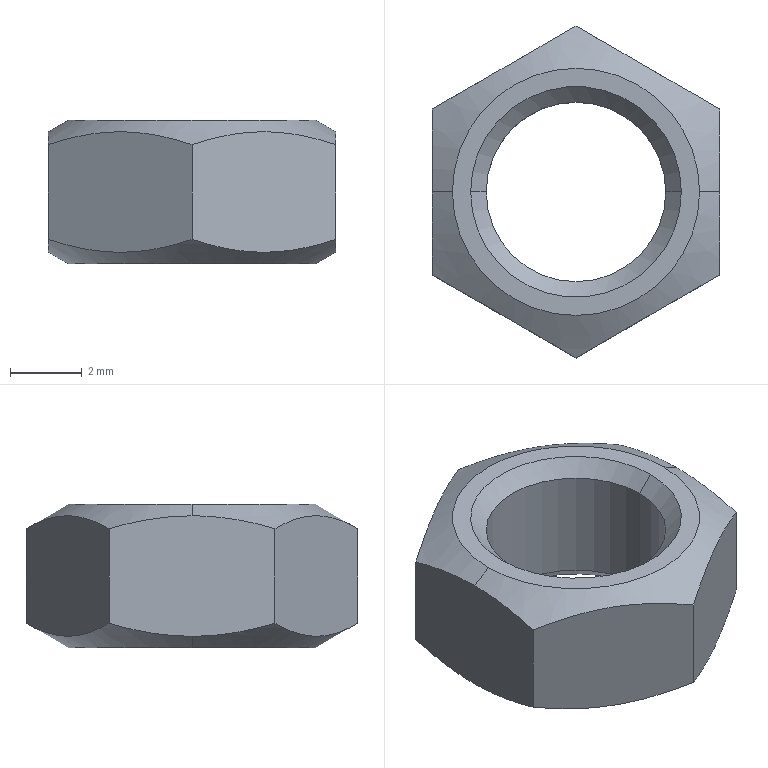Component | SolidWorks | F-YBCJ2_NTJ-015A-1 | 1 solid | 18 faces | box 8 x 9.24 x 4 mm | volume 131 mm3 | cone 8 | plane 8 | cylinder 2 | commonest cylinder face diameters 5 x2
build123d program:
from build123d import *

# Parameters (mm, degrees)
BOSS_EXTRUDE1_DEPTH      = 2
BOSS_EXTRUDE1_DEPTH_BACK = 2


with BuildPart() as part:
    # Sketch1 → Boss-Extrude1 (new, two sides: drawn at the far end of the back side and taken through both)
    with BuildSketch(Plane(origin=(0, 0, 0), x_dir=(0, 0, -1), z_dir=(1, 0, 0)).offset(-BOSS_EXTRUDE1_DEPTH_BACK)):
        Polygon((-4, 2.309), (-4, -2.309), (0, -4.619), (4, -2.309), (4, 2.309), (0, 4.619), align=None)
    extrude(amount=BOSS_EXTRUDE1_DEPTH + BOSS_EXTRUDE1_DEPTH_BACK)

    # Sketch2 → Cut-Revolve1 (revolve, cut)
    with BuildSketch(Plane.XY, mode=Mode.PRIVATE) as cut_revolve1_sk:
        Polygon((-2, 0), (-2, 2.933), (-1.567, 2.5), (1.567, 2.5), (2, 2.933), (2, 0), align=None)
    revolve(cut_revolve1_sk.sketch.rotate(Axis((2, 0, 0), (-1, 0, 0)), 270), axis=Axis((2, 0, 0), (-1, 0, 0)), mode=Mode.SUBTRACT)

    # Sketch3 → Cut-Revolve2 (revolve, cut)
    with BuildSketch(Plane.XY, mode=Mode.PRIVATE) as cut_revolve2_sk:
        Polygon((-7, 8.44), (-7, 1), (-2, 1), (-2, 3.44), (0, 6.904), (2, 3.44), (2, 1), (7, 1), (7, 8.44), align=None)
    revolve(cut_revolve2_sk.sketch.rotate(Axis((50, 0, 0), (-1, 0, 0)), 270), axis=Axis((50, 0, 0), (-1, 0, 0)), mode=Mode.SUBTRACT)


solid = part.part

# Placed as in the assembly
solid = solid.moved(Location((272.305, 302.175, 114.479), (0, 90, 0)))
STEP:
#1=COLOUR_RGB('',0.7922,0.8196,0.9333);
#2=FILL_AREA_STYLE_COLOUR('',#1);
#3=FILL_AREA_STYLE('',(#2));
#4=SURFACE_STYLE_FILL_AREA(#3);
#5=SURFACE_SIDE_STYLE('',(#4));
#6=SURFACE_STYLE_USAGE(.BOTH.,#5);
#7=PRESENTATION_STYLE_ASSIGNMENT((#6));
#8=CARTESIAN_POINT('',(10.856,11.897,4.586));
#9=VERTEX_POINT('',#8);
#10=CARTESIAN_POINT('',(10.585,11.897,4.586));
#11=VERTEX_POINT('',#10);
#12=CARTESIAN_POINT('',(10.721,11.897,4.586));
#13=DIRECTION('',(-0.,0.,1.));
#14=DIRECTION('',(1.,0.,0.));
#15=AXIS2_PLACEMENT_3D('',#12,#13,#14);
#16=CIRCLE('',#15,0.1354);
#17=EDGE_CURVE('',#9,#11,#16,.T.);
#18=ORIENTED_EDGE('',*,*,#17,.F.);
#19=CARTESIAN_POINT('',(10.878,11.897,4.573));
#20=VERTEX_POINT('',#19);
#21=CARTESIAN_POINT('',(10.856,11.897,4.586));
#22=DIRECTION('',(0.866,0.,-0.5));
#23=VECTOR('',#22,39.37);
#24=LINE('',#21,#23);
#25=EDGE_CURVE('',#9,#20,#24,.T.);
#26=ORIENTED_EDGE('',*,*,#25,.T.);
#27=CARTESIAN_POINT('',(10.878,11.988,4.559));
#28=VERTEX_POINT('',#27);
#29=CARTESIAN_POINT('',(10.878,11.897,4.573));
#30=CARTESIAN_POINT('',(10.878,11.912,4.573));
#31=CARTESIAN_POINT('',(10.878,11.928,4.572));
#32=CARTESIAN_POINT('',(10.878,11.958,4.567));
#33=CARTESIAN_POINT('',(10.878,11.973,4.563));
#34=CARTESIAN_POINT('',(10.878,11.988,4.559));
#35=B_SPLINE_CURVE_WITH_KNOTS('',3,(#29,#30,#31,#32,#33,#34),.UNSPECIFIED.,.F.,.F.,(4,2,4),(0.006456,0.007625,0.008794),.UNSPECIFIED.);
#36=EDGE_CURVE('',#20,#28,#35,.T.);
#37=ORIENTED_EDGE('',*,*,#36,.T.);
#38=CARTESIAN_POINT('',(10.721,12.079,4.559));
#39=VERTEX_POINT('',#38);
#40=CARTESIAN_POINT('',(10.878,11.988,4.559));
#41=CARTESIAN_POINT('',(10.852,12.002,4.568));
#42=CARTESIAN_POINT('',(10.826,12.018,4.573));
#43=CARTESIAN_POINT('',(10.786,12.041,4.573));
#44=CARTESIAN_POINT('',(10.773,12.048,4.572));
#45=CARTESIAN_POINT('',(10.747,12.064,4.567));
#46=CARTESIAN_POINT('',(10.734,12.071,4.563));
#47=CARTESIAN_POINT('',(10.721,12.079,4.559));
#48=B_SPLINE_CURVE_WITH_KNOTS('',3,(#40,#41,#42,#43,#44,#45,#46,#47),.UNSPECIFIED.,.F.,.F.,(4,2,2,4),(0.00000024,0.002333,0.003499,0.004665),.UNSPECIFIED.);
#49=EDGE_CURVE('',#28,#39,#48,.T.);
#50=ORIENTED_EDGE('',*,*,#49,.T.);
#51=CARTESIAN_POINT('',(10.563,11.988,4.559));
#52=VERTEX_POINT('',#51);
#53=CARTESIAN_POINT('',(10.721,12.079,4.559));
#54=CARTESIAN_POINT('',(10.695,12.064,4.568));
#55=CARTESIAN_POINT('',(10.669,12.049,4.573));
#56=CARTESIAN_POINT('',(10.629,12.025,4.573));
#57=CARTESIAN_POINT('',(10.615,12.018,4.572));
#58=CARTESIAN_POINT('',(10.589,12.003,4.567));
#59=CARTESIAN_POINT('',(10.576,11.995,4.563));
#60=CARTESIAN_POINT('',(10.563,11.988,4.559));
#61=B_SPLINE_CURVE_WITH_KNOTS('',3,(#53,#54,#55,#56,#57,#58,#59,#60),.UNSPECIFIED.,.F.,.F.,(4,2,2,4),(0.00000024,0.002333,0.003499,0.004665),.UNSPECIFIED.);
#62=EDGE_CURVE('',#39,#52,#61,.T.);
#63=ORIENTED_EDGE('',*,*,#62,.T.);
#64=CARTESIAN_POINT('',(10.563,11.897,4.573));
#65=VERTEX_POINT('',#64);
#66=CARTESIAN_POINT('',(10.563,11.988,4.559));
#67=CARTESIAN_POINT('',(10.563,11.973,4.563));
#68=CARTESIAN_POINT('',(10.563,11.958,4.567));
#69=CARTESIAN_POINT('',(10.563,11.928,4.572));
#70=CARTESIAN_POINT('',(10.563,11.912,4.573));
#71=CARTESIAN_POINT('',(10.563,11.897,4.573));
#72=B_SPLINE_CURVE_WITH_KNOTS('',3,(#66,#67,#68,#69,#70,#71),.UNSPECIFIED.,.F.,.F.,(4,2,4),(0.01181,0.01298,0.01415),.UNSPECIFIED.);
#73=EDGE_CURVE('',#52,#65,#72,.T.);
#74=ORIENTED_EDGE('',*,*,#73,.T.);
#75=CARTESIAN_POINT('',(10.585,11.897,4.586));
#76=DIRECTION('',(-0.866,0.,-0.5));
#77=VECTOR('',#76,39.37);
#78=LINE('',#75,#77);
#79=EDGE_CURVE('',#11,#65,#78,.T.);
#80=ORIENTED_EDGE('',*,*,#79,.F.);
#81=EDGE_LOOP('',(#18,#26,#37,#50,#63,#74,#80));
#82=FACE_OUTER_BOUND('',#81,.T.);
#83=CARTESIAN_POINT('',(10.721,11.897,4.586));
#84=DIRECTION('',(0.,-0.,-1.));
#85=DIRECTION('',(-1.,0.,0.));
#86=AXIS2_PLACEMENT_3D('',#83,#84,#85);
#87=CONICAL_SURFACE('',#86,0.1354,1.047);
#88=ADVANCED_FACE('',(#82),#87,.T.);
#89=CARTESIAN_POINT('',(10.856,11.897,4.428));
#90=VERTEX_POINT('',#89);
#91=CARTESIAN_POINT('',(10.585,11.897,4.428));
#92=VERTEX_POINT('',#91);
#93=CARTESIAN_POINT('',(10.721,11.897,4.428));
#94=DIRECTION('',(-0.,0.,1.));
#95=DIRECTION('',(1.,0.,0.));
#96=AXIS2_PLACEMENT_3D('',#93,#94,#95);
#97=CIRCLE('',#96,0.1354);
#98=EDGE_CURVE('',#90,#92,#97,.T.);
#99=ORIENTED_EDGE('',*,*,#98,.T.);
#100=CARTESIAN_POINT('',(10.563,11.897,4.441));
#101=VERTEX_POINT('',#100);
#102=CARTESIAN_POINT('',(10.449,11.897,4.507));
#103=DIRECTION('',(-0.866,0.,0.5));
#104=VECTOR('',#103,39.37);
#105=LINE('',#102,#104);
#106=EDGE_CURVE('',#92,#101,#105,.T.);
#107=ORIENTED_EDGE('',*,*,#106,.T.);
#108=CARTESIAN_POINT('',(10.563,11.988,4.455));
#109=VERTEX_POINT('',#108);
#110=CARTESIAN_POINT('',(10.563,11.897,4.441));
#111=CARTESIAN_POINT('',(10.563,11.912,4.441));
#112=CARTESIAN_POINT('',(10.563,11.928,4.442));
#113=CARTESIAN_POINT('',(10.563,11.958,4.447));
#114=CARTESIAN_POINT('',(10.563,11.973,4.451));
#115=CARTESIAN_POINT('',(10.563,11.988,4.455));
#116=B_SPLINE_CURVE_WITH_KNOTS('',3,(#110,#111,#112,#113,#114,#115),.UNSPECIFIED.,.F.,.F.,(4,2,4),(0.006456,0.007625,0.008794),.UNSPECIFIED.);
#117=EDGE_CURVE('',#101,#109,#116,.T.);
#118=ORIENTED_EDGE('',*,*,#117,.T.);
#119=CARTESIAN_POINT('',(10.721,12.079,4.455));
#120=VERTEX_POINT('',#119);
#121=CARTESIAN_POINT('',(10.563,11.988,4.455));
#122=CARTESIAN_POINT('',(10.589,12.002,4.447));
#123=CARTESIAN_POINT('',(10.615,12.018,4.441));
#124=CARTESIAN_POINT('',(10.655,12.041,4.441));
#125=CARTESIAN_POINT('',(10.669,12.048,4.442));
#126=CARTESIAN_POINT('',(10.695,12.064,4.447));
#127=CARTESIAN_POINT('',(10.708,12.071,4.451));
#128=CARTESIAN_POINT('',(10.721,12.079,4.455));
#129=B_SPLINE_CURVE_WITH_KNOTS('',3,(#121,#122,#123,#124,#125,#126,#127,#128),.UNSPECIFIED.,.F.,.F.,(4,2,2,4),(0.00000024,0.002333,0.003499,0.004665),.UNSPECIFIED.);
#130=EDGE_CURVE('',#109,#120,#129,.T.);
#131=ORIENTED_EDGE('',*,*,#130,.T.);
#132=CARTESIAN_POINT('',(10.878,11.988,4.455));
#133=VERTEX_POINT('',#132);
#134=CARTESIAN_POINT('',(10.721,12.079,4.455));
#135=CARTESIAN_POINT('',(10.746,12.064,4.447));
#136=CARTESIAN_POINT('',(10.772,12.049,4.441));
#137=CARTESIAN_POINT('',(10.813,12.025,4.441));
#138=CARTESIAN_POINT('',(10.826,12.018,4.442));
#139=CARTESIAN_POINT('',(10.852,12.003,4.447));
#140=CARTESIAN_POINT('',(10.865,11.995,4.451));
#141=CARTESIAN_POINT('',(10.878,11.988,4.455));
#142=B_SPLINE_CURVE_WITH_KNOTS('',3,(#134,#135,#136,#137,#138,#139,#140,#141),.UNSPECIFIED.,.F.,.F.,(4,2,2,4),(0.00000024,0.002333,0.003499,0.004665),.UNSPECIFIED.);
#143=EDGE_CURVE('',#120,#133,#142,.T.);
#144=ORIENTED_EDGE('',*,*,#143,.T.);
#145=CARTESIAN_POINT('',(10.878,11.897,4.441));
#146=VERTEX_POINT('',#145);
#147=CARTESIAN_POINT('',(10.878,11.988,4.455));
#148=CARTESIAN_POINT('',(10.878,11.973,4.451));
#149=CARTESIAN_POINT('',(10.878,11.958,4.447));
#150=CARTESIAN_POINT('',(10.878,11.928,4.442));
#151=CARTESIAN_POINT('',(10.878,11.912,4.441));
#152=CARTESIAN_POINT('',(10.878,11.897,4.441));
#153=B_SPLINE_CURVE_WITH_KNOTS('',3,(#147,#148,#149,#150,#151,#152),.UNSPECIFIED.,.F.,.F.,(4,2,4),(0.01181,0.01298,0.01415),.UNSPECIFIED.);
#154=EDGE_CURVE('',#133,#146,#153,.T.);
#155=ORIENTED_EDGE('',*,*,#154,.T.);
#156=CARTESIAN_POINT('',(10.992,11.897,4.507));
#157=DIRECTION('',(0.866,-0.,0.5));
#158=VECTOR('',#157,39.37);
#159=LINE('',#156,#158);
#160=EDGE_CURVE('',#90,#146,#159,.T.);
#161=ORIENTED_EDGE('',*,*,#160,.F.);
#162=EDGE_LOOP('',(#99,#107,#118,#131,#144,#155,#161));
#163=FACE_OUTER_BOUND('',#162,.T.);
#164=CARTESIAN_POINT('',(10.721,11.897,4.507));
#165=DIRECTION('',(-0.,0.,1.));
#166=DIRECTION('',(1.,0.,0.));
#167=AXIS2_PLACEMENT_3D('',#164,#165,#166);
#168=CONICAL_SURFACE('',#167,0.2718,1.047);
#169=ADVANCED_FACE('',(#163),#168,.T.);
#170=CARTESIAN_POINT('',(10.622,11.897,4.445));
#171=VERTEX_POINT('',#170);
#172=CARTESIAN_POINT('',(10.819,11.897,4.445));
#173=VERTEX_POINT('',#172);
#174=CARTESIAN_POINT('',(10.721,11.897,4.445));
#175=DIRECTION('',(-0.,0.,1.));
#176=DIRECTION('',(1.,0.,0.));
#177=AXIS2_PLACEMENT_3D('',#174,#175,#176);
#178=CIRCLE('',#177,0.09843);
#179=EDGE_CURVE('',#171,#173,#178,.T.);
#180=ORIENTED_EDGE('',*,*,#179,.T.);
#181=CARTESIAN_POINT('',(10.836,11.897,4.428));
#182=VERTEX_POINT('',#181);
#183=CARTESIAN_POINT('',(10.836,11.897,4.428));
#184=DIRECTION('',(0.7071,0.,-0.7071));
#185=VECTOR('',#184,39.37);
#186=LINE('',#183,#185);
#187=EDGE_CURVE('',#173,#182,#186,.T.);
#188=ORIENTED_EDGE('',*,*,#187,.T.);
#189=CARTESIAN_POINT('',(10.605,11.897,4.428));
#190=VERTEX_POINT('',#189);
#191=CARTESIAN_POINT('',(10.721,11.897,4.428));
#192=DIRECTION('',(-0.,0.,1.));
#193=DIRECTION('',(1.,0.,0.));
#194=AXIS2_PLACEMENT_3D('',#191,#192,#193);
#195=CIRCLE('',#194,0.1155);
#196=EDGE_CURVE('',#190,#182,#195,.T.);
#197=ORIENTED_EDGE('',*,*,#196,.F.);
#198=CARTESIAN_POINT('',(10.605,11.897,4.428));
#199=DIRECTION('',(-0.7071,-0.,-0.7071));
#200=VECTOR('',#199,39.37);
#201=LINE('',#198,#200);
#202=EDGE_CURVE('',#171,#190,#201,.T.);
#203=ORIENTED_EDGE('',*,*,#202,.F.);
#204=EDGE_LOOP('',(#180,#188,#197,#203));
#205=FACE_OUTER_BOUND('',#204,.T.);
#206=CARTESIAN_POINT('',(10.721,11.897,4.428));
#207=DIRECTION('',(0.,-0.,-1.));
#208=DIRECTION('',(-1.,0.,0.));
#209=AXIS2_PLACEMENT_3D('',#206,#207,#208);
#210=CONICAL_SURFACE('',#209,0.1155,0.7854);
#211=ADVANCED_FACE('',(#205),#210,.F.);
#212=ORIENTED_EDGE('',*,*,#179,.F.);
#213=CARTESIAN_POINT('',(10.622,11.897,4.569));
#214=VERTEX_POINT('',#213);
#215=CARTESIAN_POINT('',(10.622,11.897,4.428));
#216=DIRECTION('',(-0.,0.,1.));
#217=VECTOR('',#216,39.37);
#218=LINE('',#215,#217);
#219=EDGE_CURVE('',#171,#214,#218,.T.);
#220=ORIENTED_EDGE('',*,*,#219,.T.);
#221=CARTESIAN_POINT('',(10.819,11.897,4.569));
#222=VERTEX_POINT('',#221);
#223=CARTESIAN_POINT('',(10.721,11.897,4.569));
#224=DIRECTION('',(-0.,0.,1.));
#225=DIRECTION('',(1.,0.,0.));
#226=AXIS2_PLACEMENT_3D('',#223,#224,#225);
#227=CIRCLE('',#226,0.09843);
#228=EDGE_CURVE('',#214,#222,#227,.T.);
#229=ORIENTED_EDGE('',*,*,#228,.T.);
#230=CARTESIAN_POINT('',(10.819,11.897,4.428));
#231=DIRECTION('',(-0.,0.,1.));
#232=VECTOR('',#231,39.37);
#233=LINE('',#230,#232);
#234=EDGE_CURVE('',#173,#222,#233,.T.);
#235=ORIENTED_EDGE('',*,*,#234,.F.);
#236=EDGE_LOOP('',(#212,#220,#229,#235));
#237=FACE_OUTER_BOUND('',#236,.T.);
#238=CARTESIAN_POINT('',(10.721,11.897,4.428));
#239=DIRECTION('',(-0.,0.,1.));
#240=DIRECTION('',(1.,0.,0.));
#241=AXIS2_PLACEMENT_3D('',#238,#239,#240);
#242=CYLINDRICAL_SURFACE('',#241,0.09843);
#243=ADVANCED_FACE('',(#237),#242,.F.);
#244=ORIENTED_EDGE('',*,*,#228,.F.);
#245=CARTESIAN_POINT('',(10.605,11.897,4.586));
#246=VERTEX_POINT('',#245);
#247=CARTESIAN_POINT('',(10.622,11.897,4.569));
#248=DIRECTION('',(-0.7071,0.,0.7071));
#249=VECTOR('',#248,39.37);
#250=LINE('',#247,#249);
#251=EDGE_CURVE('',#214,#246,#250,.T.);
#252=ORIENTED_EDGE('',*,*,#251,.T.);
#253=CARTESIAN_POINT('',(10.836,11.897,4.586));
#254=VERTEX_POINT('',#253);
#255=CARTESIAN_POINT('',(10.721,11.897,4.586));
#256=DIRECTION('',(-0.,0.,1.));
#257=DIRECTION('',(1.,0.,0.));
#258=AXIS2_PLACEMENT_3D('',#255,#256,#257);
#259=CIRCLE('',#258,0.1155);
#260=EDGE_CURVE('',#246,#254,#259,.T.);
#261=ORIENTED_EDGE('',*,*,#260,.T.);
#262=CARTESIAN_POINT('',(10.819,11.897,4.569));
#263=DIRECTION('',(0.7071,0.,0.7071));
#264=VECTOR('',#263,39.37);
#265=LINE('',#262,#264);
#266=EDGE_CURVE('',#222,#254,#265,.T.);
#267=ORIENTED_EDGE('',*,*,#266,.F.);
#268=EDGE_LOOP('',(#244,#252,#261,#267));
#269=FACE_OUTER_BOUND('',#268,.T.);
#270=CARTESIAN_POINT('',(10.721,11.897,4.569));
#271=DIRECTION('',(-0.,0.,1.));
#272=DIRECTION('',(1.,0.,0.));
#273=AXIS2_PLACEMENT_3D('',#270,#271,#272);
#274=CONICAL_SURFACE('',#273,0.09843,0.7854);
#275=ADVANCED_FACE('',(#269),#274,.F.);
#276=ORIENTED_EDGE('',*,*,#196,.T.);
#277=CARTESIAN_POINT('',(10.721,11.897,4.428));
#278=DIRECTION('',(-0.,0.,1.));
#279=DIRECTION('',(1.,0.,0.));
#280=AXIS2_PLACEMENT_3D('',#277,#278,#279);
#281=CIRCLE('',#280,0.1155);
#282=EDGE_CURVE('',#182,#190,#281,.T.);
#283=ORIENTED_EDGE('',*,*,#282,.T.);
#284=EDGE_LOOP('',(#276,#283));
#285=FACE_BOUND('',#284,.T.);
#286=ORIENTED_EDGE('',*,*,#98,.F.);
#287=CARTESIAN_POINT('',(10.721,11.897,4.428));
#288=DIRECTION('',(-0.,0.,1.));
#289=DIRECTION('',(1.,0.,0.));
#290=AXIS2_PLACEMENT_3D('',#287,#288,#289);
#291=CIRCLE('',#290,0.1354);
#292=EDGE_CURVE('',#92,#90,#291,.T.);
#293=ORIENTED_EDGE('',*,*,#292,.F.);
#294=EDGE_LOOP('',(#286,#293));
#295=FACE_OUTER_BOUND('',#294,.T.);
#296=CARTESIAN_POINT('',(10.721,11.897,4.428));
#297=DIRECTION('',(0.,-0.,-1.));
#298=DIRECTION('',(-1.,0.,-0.));
#299=AXIS2_PLACEMENT_3D('',#296,#297,#298);
#300=PLANE('',#299);
#301=ADVANCED_FACE('',(#285,#295),#300,.T.);
#302=CARTESIAN_POINT('',(10.721,11.897,4.586));
#303=DIRECTION('',(-0.,0.,1.));
#304=DIRECTION('',(1.,0.,0.));
#305=AXIS2_PLACEMENT_3D('',#302,#303,#304);
#306=CIRCLE('',#305,0.1155);
#307=EDGE_CURVE('',#254,#246,#306,.T.);
#308=ORIENTED_EDGE('',*,*,#307,.F.);
#309=ORIENTED_EDGE('',*,*,#260,.F.);
#310=EDGE_LOOP('',(#308,#309));
#311=FACE_BOUND('',#310,.T.);
#312=CARTESIAN_POINT('',(10.721,11.897,4.586));
#313=DIRECTION('',(-0.,0.,1.));
#314=DIRECTION('',(1.,0.,0.));
#315=AXIS2_PLACEMENT_3D('',#312,#313,#314);
#316=CIRCLE('',#315,0.1354);
#317=EDGE_CURVE('',#11,#9,#316,.T.);
#318=ORIENTED_EDGE('',*,*,#317,.T.);
#319=ORIENTED_EDGE('',*,*,#17,.T.);
#320=EDGE_LOOP('',(#318,#319));
#321=FACE_OUTER_BOUND('',#320,.T.);
#322=CARTESIAN_POINT('',(10.721,11.897,4.586));
#323=DIRECTION('',(0.,-0.,-1.));
#324=DIRECTION('',(-1.,0.,-0.));
#325=AXIS2_PLACEMENT_3D('',#322,#323,#324);
#326=PLANE('',#325);
#327=ADVANCED_FACE('',(#311,#321),#326,.F.);
#328=ORIENTED_EDGE('',*,*,#251,.F.);
#329=CARTESIAN_POINT('',(10.721,11.897,4.569));
#330=DIRECTION('',(-0.,0.,1.));
#331=DIRECTION('',(1.,0.,0.));
#332=AXIS2_PLACEMENT_3D('',#329,#330,#331);
#333=CIRCLE('',#332,0.09843);
#334=EDGE_CURVE('',#222,#214,#333,.T.);
#335=ORIENTED_EDGE('',*,*,#334,.F.);
#336=ORIENTED_EDGE('',*,*,#266,.T.);
#337=ORIENTED_EDGE('',*,*,#307,.T.);
#338=EDGE_LOOP('',(#328,#335,#336,#337));
#339=FACE_OUTER_BOUND('',#338,.T.);
#340=CARTESIAN_POINT('',(10.721,11.897,4.569));
#341=DIRECTION('',(-0.,0.,1.));
#342=DIRECTION('',(1.,0.,0.));
#343=AXIS2_PLACEMENT_3D('',#340,#341,#342);
#344=CONICAL_SURFACE('',#343,0.09843,0.7854);
#345=ADVANCED_FACE('',(#339),#344,.F.);
#346=ORIENTED_EDGE('',*,*,#219,.F.);
#347=CARTESIAN_POINT('',(10.721,11.897,4.445));
#348=DIRECTION('',(-0.,0.,1.));
#349=DIRECTION('',(1.,0.,0.));
#350=AXIS2_PLACEMENT_3D('',#347,#348,#349);
#351=CIRCLE('',#350,0.09843);
#352=EDGE_CURVE('',#173,#171,#351,.T.);
#353=ORIENTED_EDGE('',*,*,#352,.F.);
#354=ORIENTED_EDGE('',*,*,#234,.T.);
#355=ORIENTED_EDGE('',*,*,#334,.T.);
#356=EDGE_LOOP('',(#346,#353,#354,#355));
#357=FACE_OUTER_BOUND('',#356,.T.);
#358=CARTESIAN_POINT('',(10.721,11.897,4.428));
#359=DIRECTION('',(-0.,0.,1.));
#360=DIRECTION('',(1.,0.,0.));
#361=AXIS2_PLACEMENT_3D('',#358,#359,#360);
#362=CYLINDRICAL_SURFACE('',#361,0.09843);
#363=ADVANCED_FACE('',(#357),#362,.F.);
#364=ORIENTED_EDGE('',*,*,#187,.F.);
#365=ORIENTED_EDGE('',*,*,#352,.T.);
#366=ORIENTED_EDGE('',*,*,#202,.T.);
#367=ORIENTED_EDGE('',*,*,#282,.F.);
#368=EDGE_LOOP('',(#364,#365,#366,#367));
#369=FACE_OUTER_BOUND('',#368,.T.);
#370=CARTESIAN_POINT('',(10.721,11.897,4.428));
#371=DIRECTION('',(0.,-0.,-1.));
#372=DIRECTION('',(-1.,0.,0.));
#373=AXIS2_PLACEMENT_3D('',#370,#371,#372);
#374=CONICAL_SURFACE('',#373,0.1155,0.7854);
#375=ADVANCED_FACE('',(#369),#374,.F.);
#376=ORIENTED_EDGE('',*,*,#106,.F.);
#377=ORIENTED_EDGE('',*,*,#292,.T.);
#378=ORIENTED_EDGE('',*,*,#160,.T.);
#379=CARTESIAN_POINT('',(10.878,11.806,4.455));
#380=VERTEX_POINT('',#379);
#381=CARTESIAN_POINT('',(10.878,11.897,4.441));
#382=CARTESIAN_POINT('',(10.878,11.881,4.441));
#383=CARTESIAN_POINT('',(10.878,11.866,4.442));
#384=CARTESIAN_POINT('',(10.878,11.836,4.447));
#385=CARTESIAN_POINT('',(10.878,11.821,4.451));
#386=CARTESIAN_POINT('',(10.878,11.806,4.455));
#387=B_SPLINE_CURVE_WITH_KNOTS('',3,(#381,#382,#383,#384,#385,#386),.UNSPECIFIED.,.F.,.F.,(4,2,4),(0.01415,0.01532,0.01649),.UNSPECIFIED.);
#388=EDGE_CURVE('',#146,#380,#387,.T.);
#389=ORIENTED_EDGE('',*,*,#388,.T.);
#390=CARTESIAN_POINT('',(10.721,11.715,4.455));
#391=VERTEX_POINT('',#390);
#392=CARTESIAN_POINT('',(10.878,11.806,4.455));
#393=CARTESIAN_POINT('',(10.852,11.791,4.447));
#394=CARTESIAN_POINT('',(10.826,11.776,4.441));
#395=CARTESIAN_POINT('',(10.786,11.753,4.441));
#396=CARTESIAN_POINT('',(10.773,11.745,4.442));
#397=CARTESIAN_POINT('',(10.747,11.73,4.447));
#398=CARTESIAN_POINT('',(10.734,11.722,4.451));
#399=CARTESIAN_POINT('',(10.721,11.715,4.455));
#400=B_SPLINE_CURVE_WITH_KNOTS('',3,(#392,#393,#394,#395,#396,#397,#398,#399),.UNSPECIFIED.,.F.,.F.,(4,2,2,4),(0.00000024,0.002333,0.003499,0.004665),.UNSPECIFIED.);
#401=EDGE_CURVE('',#380,#391,#400,.T.);
#402=ORIENTED_EDGE('',*,*,#401,.T.);
#403=CARTESIAN_POINT('',(10.563,11.806,4.455));
#404=VERTEX_POINT('',#403);
#405=CARTESIAN_POINT('',(10.721,11.715,4.455));
#406=CARTESIAN_POINT('',(10.695,11.73,4.447));
#407=CARTESIAN_POINT('',(10.669,11.745,4.441));
#408=CARTESIAN_POINT('',(10.629,11.768,4.441));
#409=CARTESIAN_POINT('',(10.615,11.776,4.442));
#410=CARTESIAN_POINT('',(10.589,11.791,4.447));
#411=CARTESIAN_POINT('',(10.576,11.798,4.451));
#412=CARTESIAN_POINT('',(10.563,11.806,4.455));
#413=B_SPLINE_CURVE_WITH_KNOTS('',3,(#405,#406,#407,#408,#409,#410,#411,#412),.UNSPECIFIED.,.F.,.F.,(4,2,2,4),(0.00000024,0.002333,0.003499,0.004665),.UNSPECIFIED.);
#414=EDGE_CURVE('',#391,#404,#413,.T.);
#415=ORIENTED_EDGE('',*,*,#414,.T.);
#416=CARTESIAN_POINT('',(10.563,11.806,4.455));
#417=CARTESIAN_POINT('',(10.563,11.821,4.451));
#418=CARTESIAN_POINT('',(10.563,11.836,4.447));
#419=CARTESIAN_POINT('',(10.563,11.866,4.442));
#420=CARTESIAN_POINT('',(10.563,11.881,4.441));
#421=CARTESIAN_POINT('',(10.563,11.897,4.441));
#422=B_SPLINE_CURVE_WITH_KNOTS('',3,(#416,#417,#418,#419,#420,#421),.UNSPECIFIED.,.F.,.F.,(4,2,4),(0.00412,0.005288,0.006456),.UNSPECIFIED.);
#423=EDGE_CURVE('',#404,#101,#422,.T.);
#424=ORIENTED_EDGE('',*,*,#423,.T.);
#425=EDGE_LOOP('',(#376,#377,#378,#389,#402,#415,#424));
#426=FACE_OUTER_BOUND('',#425,.T.);
#427=CARTESIAN_POINT('',(10.721,11.897,4.507));
#428=DIRECTION('',(-0.,0.,1.));
#429=DIRECTION('',(1.,0.,0.));
#430=AXIS2_PLACEMENT_3D('',#427,#428,#429);
#431=CONICAL_SURFACE('',#430,0.2718,1.047);
#432=ADVANCED_FACE('',(#426),#431,.T.);
#433=ORIENTED_EDGE('',*,*,#25,.F.);
#434=ORIENTED_EDGE('',*,*,#317,.F.);
#435=ORIENTED_EDGE('',*,*,#79,.T.);
#436=CARTESIAN_POINT('',(10.563,11.806,4.559));
#437=VERTEX_POINT('',#436);
#438=CARTESIAN_POINT('',(10.563,11.897,4.573));
#439=CARTESIAN_POINT('',(10.563,11.881,4.573));
#440=CARTESIAN_POINT('',(10.563,11.866,4.572));
#441=CARTESIAN_POINT('',(10.563,11.836,4.567));
#442=CARTESIAN_POINT('',(10.563,11.821,4.563));
#443=CARTESIAN_POINT('',(10.563,11.806,4.559));
#444=B_SPLINE_CURVE_WITH_KNOTS('',3,(#438,#439,#440,#441,#442,#443),.UNSPECIFIED.,.F.,.F.,(4,2,4),(0.01415,0.01532,0.01649),.UNSPECIFIED.);
#445=EDGE_CURVE('',#65,#437,#444,.T.);
#446=ORIENTED_EDGE('',*,*,#445,.T.);
#447=CARTESIAN_POINT('',(10.721,11.715,4.559));
#448=VERTEX_POINT('',#447);
#449=CARTESIAN_POINT('',(10.563,11.806,4.559));
#450=CARTESIAN_POINT('',(10.589,11.791,4.568));
#451=CARTESIAN_POINT('',(10.615,11.776,4.573));
#452=CARTESIAN_POINT('',(10.655,11.753,4.573));
#453=CARTESIAN_POINT('',(10.669,11.745,4.572));
#454=CARTESIAN_POINT('',(10.695,11.73,4.567));
#455=CARTESIAN_POINT('',(10.708,11.722,4.563));
#456=CARTESIAN_POINT('',(10.721,11.715,4.559));
#457=B_SPLINE_CURVE_WITH_KNOTS('',3,(#449,#450,#451,#452,#453,#454,#455,#456),.UNSPECIFIED.,.F.,.F.,(4,2,2,4),(0.00000024,0.002333,0.003499,0.004665),.UNSPECIFIED.);
#458=EDGE_CURVE('',#437,#448,#457,.T.);
#459=ORIENTED_EDGE('',*,*,#458,.T.);
#460=CARTESIAN_POINT('',(10.878,11.806,4.559));
#461=VERTEX_POINT('',#460);
#462=CARTESIAN_POINT('',(10.721,11.715,4.559));
#463=CARTESIAN_POINT('',(10.746,11.73,4.568));
#464=CARTESIAN_POINT('',(10.772,11.745,4.573));
#465=CARTESIAN_POINT('',(10.813,11.768,4.573));
#466=CARTESIAN_POINT('',(10.826,11.776,4.572));
#467=CARTESIAN_POINT('',(10.852,11.791,4.567));
#468=CARTESIAN_POINT('',(10.865,11.798,4.563));
#469=CARTESIAN_POINT('',(10.878,11.806,4.559));
#470=B_SPLINE_CURVE_WITH_KNOTS('',3,(#462,#463,#464,#465,#466,#467,#468,#469),.UNSPECIFIED.,.F.,.F.,(4,2,2,4),(0.00000024,0.002333,0.003499,0.004665),.UNSPECIFIED.);
#471=EDGE_CURVE('',#448,#461,#470,.T.);
#472=ORIENTED_EDGE('',*,*,#471,.T.);
#473=CARTESIAN_POINT('',(10.878,11.806,4.559));
#474=CARTESIAN_POINT('',(10.878,11.821,4.563));
#475=CARTESIAN_POINT('',(10.878,11.836,4.567));
#476=CARTESIAN_POINT('',(10.878,11.866,4.572));
#477=CARTESIAN_POINT('',(10.878,11.881,4.573));
#478=CARTESIAN_POINT('',(10.878,11.897,4.573));
#479=B_SPLINE_CURVE_WITH_KNOTS('',3,(#473,#474,#475,#476,#477,#478),.UNSPECIFIED.,.F.,.F.,(4,2,4),(0.00412,0.005288,0.006456),.UNSPECIFIED.);
#480=EDGE_CURVE('',#461,#20,#479,.T.);
#481=ORIENTED_EDGE('',*,*,#480,.T.);
#482=EDGE_LOOP('',(#433,#434,#435,#446,#459,#472,#481));
#483=FACE_OUTER_BOUND('',#482,.T.);
#484=CARTESIAN_POINT('',(10.721,11.897,4.586));
#485=DIRECTION('',(0.,-0.,-1.));
#486=DIRECTION('',(-1.,0.,0.));
#487=AXIS2_PLACEMENT_3D('',#484,#485,#486);
#488=CONICAL_SURFACE('',#487,0.1354,1.047);
#489=ADVANCED_FACE('',(#483),#488,.T.);
#490=ORIENTED_EDGE('',*,*,#62,.F.);
#491=CARTESIAN_POINT('',(10.721,12.079,4.428));
#492=DIRECTION('',(-0.,0.,1.));
#493=VECTOR('',#492,39.37);
#494=LINE('',#491,#493);
#495=EDGE_CURVE('',#120,#39,#494,.T.);
#496=ORIENTED_EDGE('',*,*,#495,.F.);
#497=ORIENTED_EDGE('',*,*,#130,.F.);
#498=CARTESIAN_POINT('',(10.563,11.988,4.428));
#499=DIRECTION('',(-0.,0.,1.));
#500=VECTOR('',#499,39.37);
#501=LINE('',#498,#500);
#502=EDGE_CURVE('',#109,#52,#501,.T.);
#503=ORIENTED_EDGE('',*,*,#502,.T.);
#504=EDGE_LOOP('',(#490,#496,#497,#503));
#505=FACE_OUTER_BOUND('',#504,.T.);
#506=CARTESIAN_POINT('',(10.563,11.988,4.428));
#507=DIRECTION('',(0.5,-0.866,0.));
#508=DIRECTION('',(-0.866,-0.5,-0.));
#509=AXIS2_PLACEMENT_3D('',#506,#507,#508);
#510=PLANE('',#509);
#511=ADVANCED_FACE('',(#505),#510,.F.);
#512=ORIENTED_EDGE('',*,*,#73,.F.);
#513=ORIENTED_EDGE('',*,*,#502,.F.);
#514=ORIENTED_EDGE('',*,*,#117,.F.);
#515=ORIENTED_EDGE('',*,*,#423,.F.);
#516=CARTESIAN_POINT('',(10.563,11.806,4.428));
#517=DIRECTION('',(-0.,0.,1.));
#518=VECTOR('',#517,39.37);
#519=LINE('',#516,#518);
#520=EDGE_CURVE('',#404,#437,#519,.T.);
#521=ORIENTED_EDGE('',*,*,#520,.T.);
#522=ORIENTED_EDGE('',*,*,#445,.F.);
#523=EDGE_LOOP('',(#512,#513,#514,#515,#521,#522));
#524=FACE_OUTER_BOUND('',#523,.T.);
#525=CARTESIAN_POINT('',(10.563,11.806,4.428));
#526=DIRECTION('',(1.,-0.,0.));
#527=DIRECTION('',(0.,-0.,-1.));
#528=AXIS2_PLACEMENT_3D('',#525,#526,#527);
#529=PLANE('',#528);
#530=ADVANCED_FACE('',(#524),#529,.F.);
#531=ORIENTED_EDGE('',*,*,#458,.F.);
#532=ORIENTED_EDGE('',*,*,#520,.F.);
#533=ORIENTED_EDGE('',*,*,#414,.F.);
#534=CARTESIAN_POINT('',(10.721,11.715,4.428));
#535=DIRECTION('',(-0.,0.,1.));
#536=VECTOR('',#535,39.37);
#537=LINE('',#534,#536);
#538=EDGE_CURVE('',#391,#448,#537,.T.);
#539=ORIENTED_EDGE('',*,*,#538,.T.);
#540=EDGE_LOOP('',(#531,#532,#533,#539));
#541=FACE_OUTER_BOUND('',#540,.T.);
#542=CARTESIAN_POINT('',(10.721,11.715,4.428));
#543=DIRECTION('',(0.5,0.866,0.));
#544=DIRECTION('',(0.866,-0.5,0.));
#545=AXIS2_PLACEMENT_3D('',#542,#543,#544);
#546=PLANE('',#545);
#547=ADVANCED_FACE('',(#541),#546,.F.);
#548=ORIENTED_EDGE('',*,*,#471,.F.);
#549=ORIENTED_EDGE('',*,*,#538,.F.);
#550=ORIENTED_EDGE('',*,*,#401,.F.);
#551=CARTESIAN_POINT('',(10.878,11.806,4.428));
#552=DIRECTION('',(-0.,0.,1.));
#553=VECTOR('',#552,39.37);
#554=LINE('',#551,#553);
#555=EDGE_CURVE('',#380,#461,#554,.T.);
#556=ORIENTED_EDGE('',*,*,#555,.T.);
#557=EDGE_LOOP('',(#548,#549,#550,#556));
#558=FACE_OUTER_BOUND('',#557,.T.);
#559=CARTESIAN_POINT('',(10.878,11.806,4.428));
#560=DIRECTION('',(-0.5,0.866,-0.));
#561=DIRECTION('',(0.866,0.5,0.));
#562=AXIS2_PLACEMENT_3D('',#559,#560,#561);
#563=PLANE('',#562);
#564=ADVANCED_FACE('',(#558),#563,.F.);
#565=ORIENTED_EDGE('',*,*,#480,.F.);
#566=ORIENTED_EDGE('',*,*,#555,.F.);
#567=ORIENTED_EDGE('',*,*,#388,.F.);
#568=ORIENTED_EDGE('',*,*,#154,.F.);
#569=CARTESIAN_POINT('',(10.878,11.988,4.428));
#570=DIRECTION('',(-0.,0.,1.));
#571=VECTOR('',#570,39.37);
#572=LINE('',#569,#571);
#573=EDGE_CURVE('',#133,#28,#572,.T.);
#574=ORIENTED_EDGE('',*,*,#573,.T.);
#575=ORIENTED_EDGE('',*,*,#36,.F.);
#576=EDGE_LOOP('',(#565,#566,#567,#568,#574,#575));
#577=FACE_OUTER_BOUND('',#576,.T.);
#578=CARTESIAN_POINT('',(10.878,11.988,4.428));
#579=DIRECTION('',(-1.,0.,-0.));
#580=DIRECTION('',(-0.,0.,1.));
#581=AXIS2_PLACEMENT_3D('',#578,#579,#580);
#582=PLANE('',#581);
#583=ADVANCED_FACE('',(#577),#582,.F.);
#584=ORIENTED_EDGE('',*,*,#49,.F.);
#585=ORIENTED_EDGE('',*,*,#573,.F.);
#586=ORIENTED_EDGE('',*,*,#143,.F.);
#587=ORIENTED_EDGE('',*,*,#495,.T.);
#588=EDGE_LOOP('',(#584,#585,#586,#587));
#589=FACE_OUTER_BOUND('',#588,.T.);
#590=CARTESIAN_POINT('',(10.721,12.079,4.428));
#591=DIRECTION('',(-0.5,-0.866,-0.));
#592=DIRECTION('',(-0.866,0.5,-0.));
#593=AXIS2_PLACEMENT_3D('',#590,#591,#592);
#594=PLANE('',#593);
#595=ADVANCED_FACE('',(#589),#594,.F.);
#596=CLOSED_SHELL('',(#88,#169,#211,#243,#275,#301,#327,#345,#363,#375,#432,#489,#511,#530,#547,#564,#583,#595));
#597=MANIFOLD_SOLID_BREP('',#596);
#598=STYLED_ITEM('',(#7),#597);
#599=PRESENTATION_LAYER_ASSIGNMENT('','',(#598));
#600=(LENGTH_UNIT()NAMED_UNIT(*)SI_UNIT($,.METRE.));
#601=LENGTH_MEASURE_WITH_UNIT(LENGTH_MEASURE(0.0254),#600);
#602=DIMENSIONAL_EXPONENTS(1.,0.,0.,0.,0.,0.,0.);
#603=(CONVERSION_BASED_UNIT('',#601)LENGTH_UNIT()NAMED_UNIT(#602));
#604=UNCERTAINTY_MEASURE_WITH_UNIT(LENGTH_MEASURE(0.00001),#603,'','');
#605=(NAMED_UNIT(*)PLANE_ANGLE_UNIT()SI_UNIT($,.RADIAN.));
#606=(NAMED_UNIT(*)SI_UNIT($,.STERADIAN.)SOLID_ANGLE_UNIT());
#607=(GEOMETRIC_REPRESENTATION_CONTEXT(3)GLOBAL_UNCERTAINTY_ASSIGNED_CONTEXT((#604))GLOBAL_UNIT_ASSIGNED_CONTEXT((#603,#605,#606))REPRESENTATION_CONTEXT('',''));
#608=MECHANICAL_DESIGN_GEOMETRIC_PRESENTATION_REPRESENTATION('',(#598),#607);
#609=CARTESIAN_POINT('',(0.,0.,0.));
#610=DIRECTION('',(0.,0.,1.));
#611=DIRECTION('',(1.,0.,0.));
#612=AXIS2_PLACEMENT_3D('',#609,#610,#611);
#613=(LENGTH_UNIT()NAMED_UNIT(*)SI_UNIT($,.METRE.));
#614=LENGTH_MEASURE_WITH_UNIT(LENGTH_MEASURE(0.0254),#613);
#615=DIMENSIONAL_EXPONENTS(1.,0.,0.,0.,0.,0.,0.);
#616=(CONVERSION_BASED_UNIT('',#614)LENGTH_UNIT()NAMED_UNIT(#615));
#617=UNCERTAINTY_MEASURE_WITH_UNIT(LENGTH_MEASURE(0.00001),#616,'','');
#618=(NAMED_UNIT(*)PLANE_ANGLE_UNIT()SI_UNIT($,.RADIAN.));
#619=(NAMED_UNIT(*)SI_UNIT($,.STERADIAN.)SOLID_ANGLE_UNIT());
#620=(GEOMETRIC_REPRESENTATION_CONTEXT(3)GLOBAL_UNCERTAINTY_ASSIGNED_CONTEXT((#617))GLOBAL_UNIT_ASSIGNED_CONTEXT((#616,#618,#619))REPRESENTATION_CONTEXT('',''));
#621=ADVANCED_BREP_SHAPE_REPRESENTATION('',(#597,#612),#620);